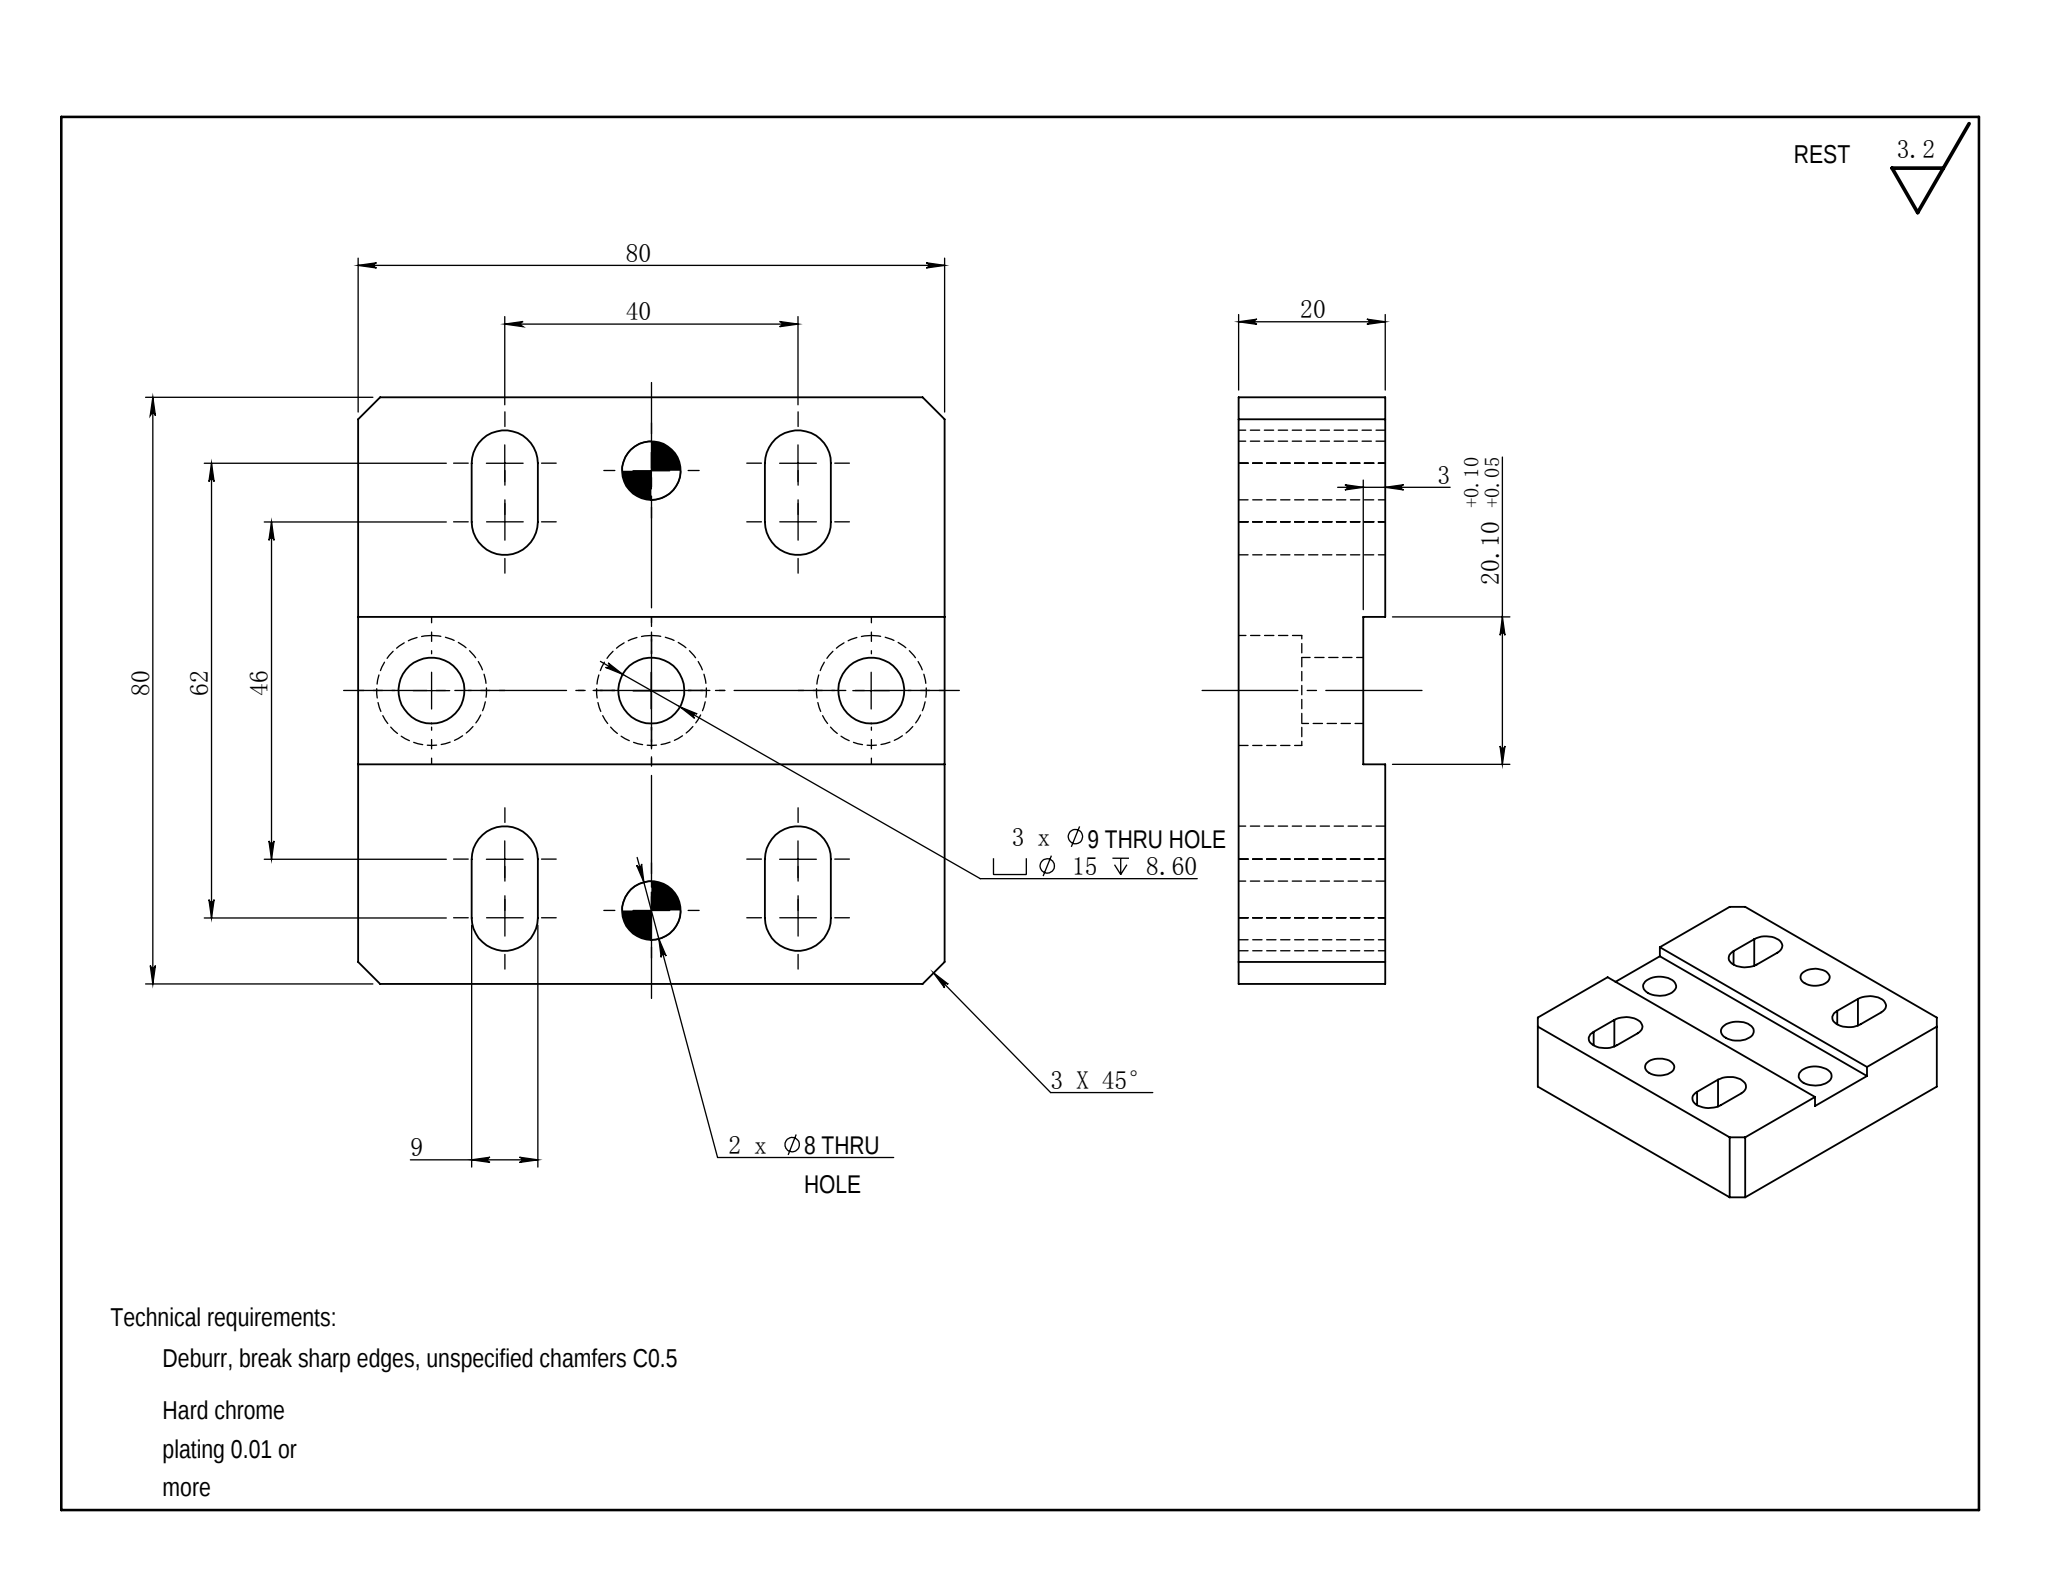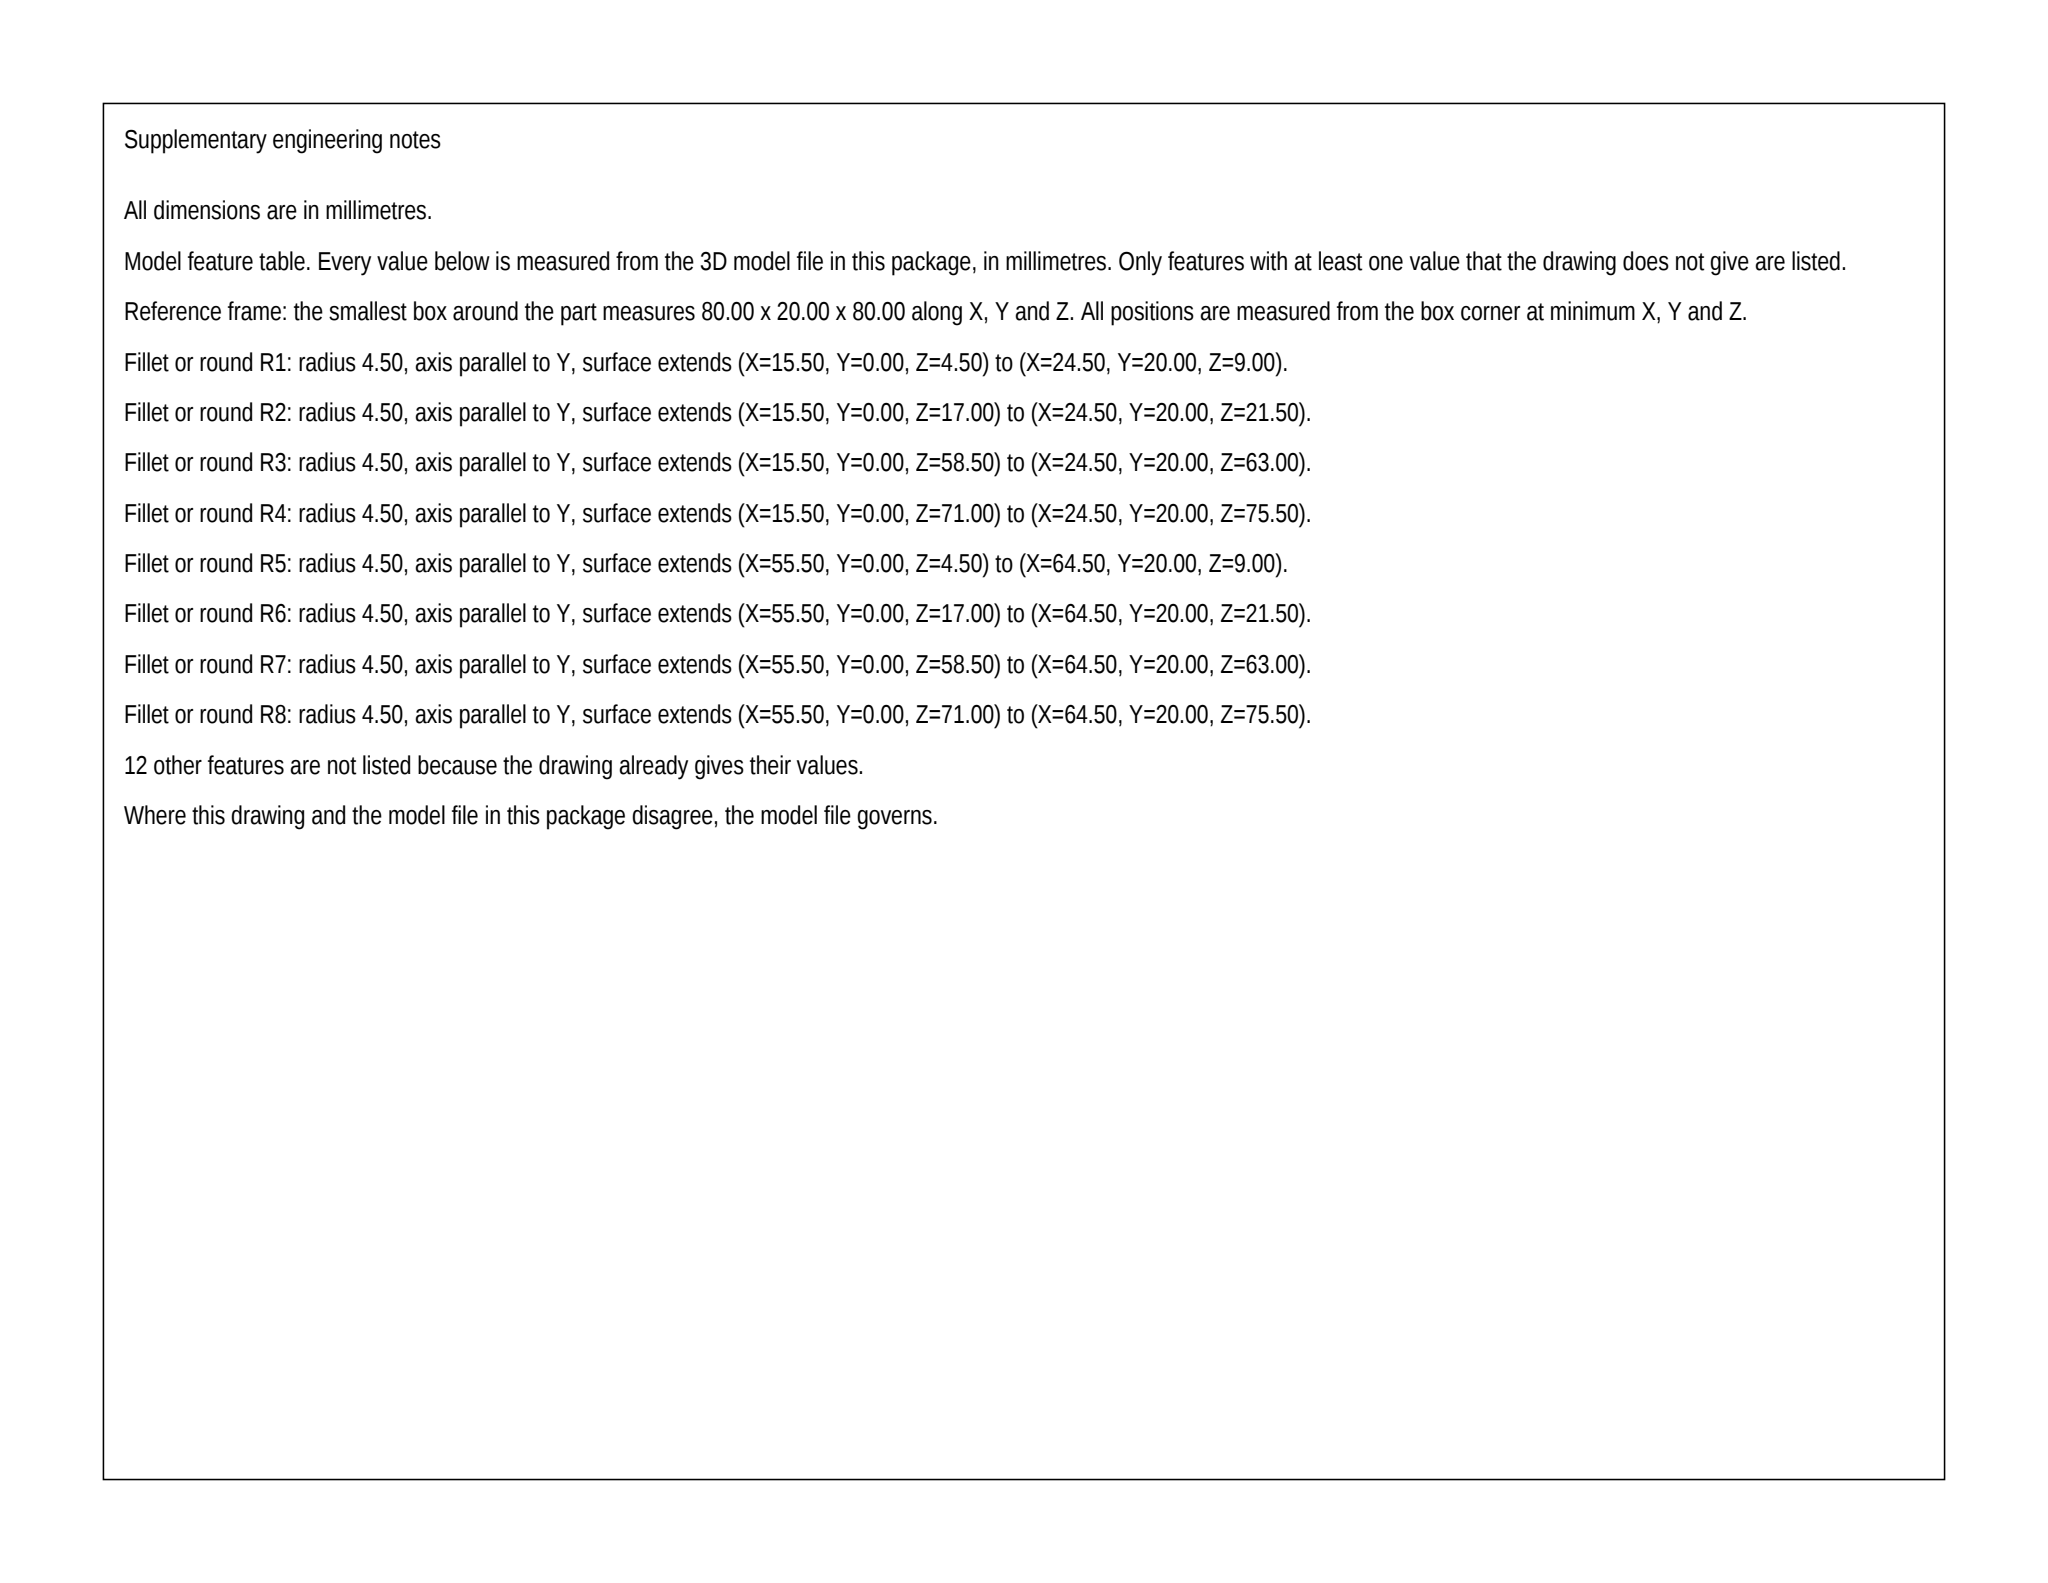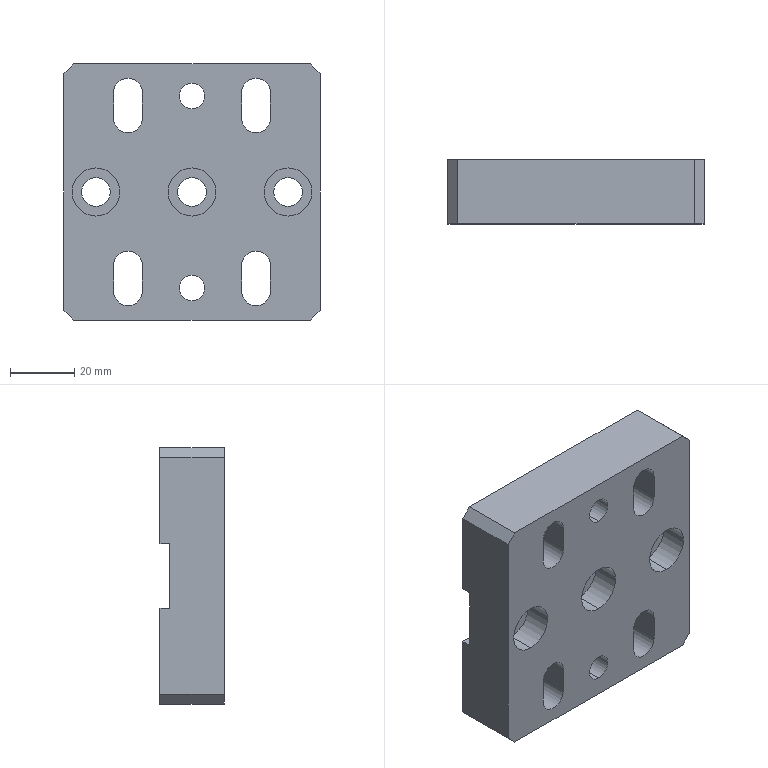Part | SolidWorks | mm | 1 solid | 53 faces | box 80 x 20 x 80 mm | volume 103794 mm3 | cylinder 28 | plane 25 | commonest cylinder face diameters 9 x18 15 x6 8 x4
Drawing notes:
RECESS BAND 20.10 WIDE x 3 DP, SYM ABOUT HORIZ CL (CL 40 FROM EDGE) | from the solid: z-planes 29.95 & 50.05 = 20.10 band ctrd on z=40; y-planes 17 & 20 give 3 deep step
4 SLOTS Ø9 THRU, 9 WIDE x 17 OAL, R4.5 ENDS, 8 C/C; SLOT CL AT X=20 & 60 | from the solid: Ø9 y-cyls L=20 paired z=9/17 & z=63/71 at x=20,60; x-planes 15.5/24.5 & 55.5/64.5
2 x Ø8 THRU ON VERT CL, 60 C/C, 10 FROM TOP & BOT EDGES | from the solid: Ø8 y-cyls L=20 at x=40, z=10 and z=70 in 80 x 80 bbox
3 x Ø9 THRU ON HORIZ CL, 30 C/C, 10 FROM EA SIDE | from the solid: Ø9/Ø15 cyls at x=10, 40, 70, z=40, bbox X=80
CBORE Ø15 DP 8.60 FROM BACK FACE; Ø9 REM 8.40 BREAKS INTO RECESS FACE | from the solid: Ø15 L=8.6 and Ø9 L=8.4 at z=40; y-planes 0, 8.6, 17 (8.60+8.40=17)
build123d program:
from build123d import *

# Parameters (mm, degrees)
SKETCH1_W                                       = 80
SKETCH1_H                                       = 80
BOSS_EXTRUDE1_DEPTH                             = 10
CHAMFER1_SIZE                                   = 3
SKETCH2_W                                       = 80
SKETCH2_H                                       = 20.1
CUT_EXTRUDE1_DEPTH                              = 3
F_9_0_9_DIAMETER_HOLE1_D                        = 9
M8_HEX_SOCKET_HEAD_CAP_SCREW_CBORE1_D           = 9
M8_HEX_SOCKET_HEAD_CAP_SCREW_CBORE1_CBORE_D     = 15
M8_HEX_SOCKET_HEAD_CAP_SCREW_CBORE1_CBORE_DEPTH = 8.6
CUT_EXTRUDE2_DEPTH                              = 61
F_8_0_8_DIAMETER_HOLE1_D                        = 8


with BuildPart() as part:
    # Sketch1 → Boss-Extrude1 (new, symmetric)
    with BuildSketch(Plane(origin=(0, 0, 0), x_dir=(1, 0, 0), z_dir=(0, 1, 0))):
        Rectangle(SKETCH1_W, SKETCH1_H)
    extrude(amount=BOSS_EXTRUDE1_DEPTH, both=True)

    # Chamfer1
    chamfer1_edges = [part.edges().sort_by_distance(p)[0] for p in [
        (40, 0, 40),
        (-40, 0, 40),
        (-40, 0, -40),
        (40, 0, -40),
    ]]
    chamfer(chamfer1_edges, length=CHAMFER1_SIZE)

    # Sketch2 → Cut-Extrude1 (cut)
    with BuildSketch(Plane(origin=(0, 10, 0), x_dir=(1, 0, 0), z_dir=(0, 1, 0))):
        Rectangle(SKETCH2_W, SKETCH2_H)
    extrude(amount=-CUT_EXTRUDE1_DEPTH, mode=Mode.SUBTRACT)

    # 9.0 _9_ Diameter Hole1 (through all)
    with Locations(Plane(origin=(0, 10, 0), x_dir=(1, 0, 0), z_dir=(0, 1, 0))):
        with Locations((-20, 27), (-20, -27), (20, 27), (20, -27)):
            Hole(F_9_0_9_DIAMETER_HOLE1_D / 2)

    # M8 Hex Socket Head Cap Screw CBORE1 (through all)
    with Locations(Plane(origin=(0, -10, 0), x_dir=(-1, 0, 0), z_dir=(0, -1, 0))):
        with Locations((0, 0), (-30, 0), (30, 0)):
            CounterBoreHole(M8_HEX_SOCKET_HEAD_CAP_SCREW_CBORE1_D / 2, M8_HEX_SOCKET_HEAD_CAP_SCREW_CBORE1_CBORE_D / 2, M8_HEX_SOCKET_HEAD_CAP_SCREW_CBORE1_CBORE_DEPTH)

    # Sketch11 → Cut-Extrude2 (cut, through all)
    with BuildSketch(Plane(origin=(0, 10, 0), x_dir=(1, 0, 0), z_dir=(0, 1, 0))):
        with BuildLine():
            Line((-24.5, 23), (-24.5, 31))
            ThreePointArc((-24.5, 31), (-20, 35.5), (-15.5, 31))
            Line((-15.5, 31), (-15.5, 23))
            ThreePointArc((-15.5, 23), (-20, 18.5), (-24.5, 23))
        make_face()
        with BuildLine():
            Line((15.5, 23), (15.5, 31))
            ThreePointArc((15.5, 31), (20, 35.5), (24.5, 31))
            Line((24.5, 31), (24.5, 23))
            ThreePointArc((24.5, 23), (20, 18.5), (15.5, 23))
        make_face()
    cut_extrude2 = extrude(amount=-CUT_EXTRUDE2_DEPTH, mode=Mode.SUBTRACT)

    # Mirror1: Cut-Extrude2 across plane
    add(cut_extrude2.mirror(Plane.XY), mode=Mode.SUBTRACT)

    # 8.0 _8_ Diameter Hole1 (through all)
    with Locations(Plane(origin=(0, 10, 0), x_dir=(1, 0, 0), z_dir=(0, 1, 0))):
        with Locations((0, 30), (0, -30)):
            Hole(F_8_0_8_DIAMETER_HOLE1_D / 2)


solid = part.part